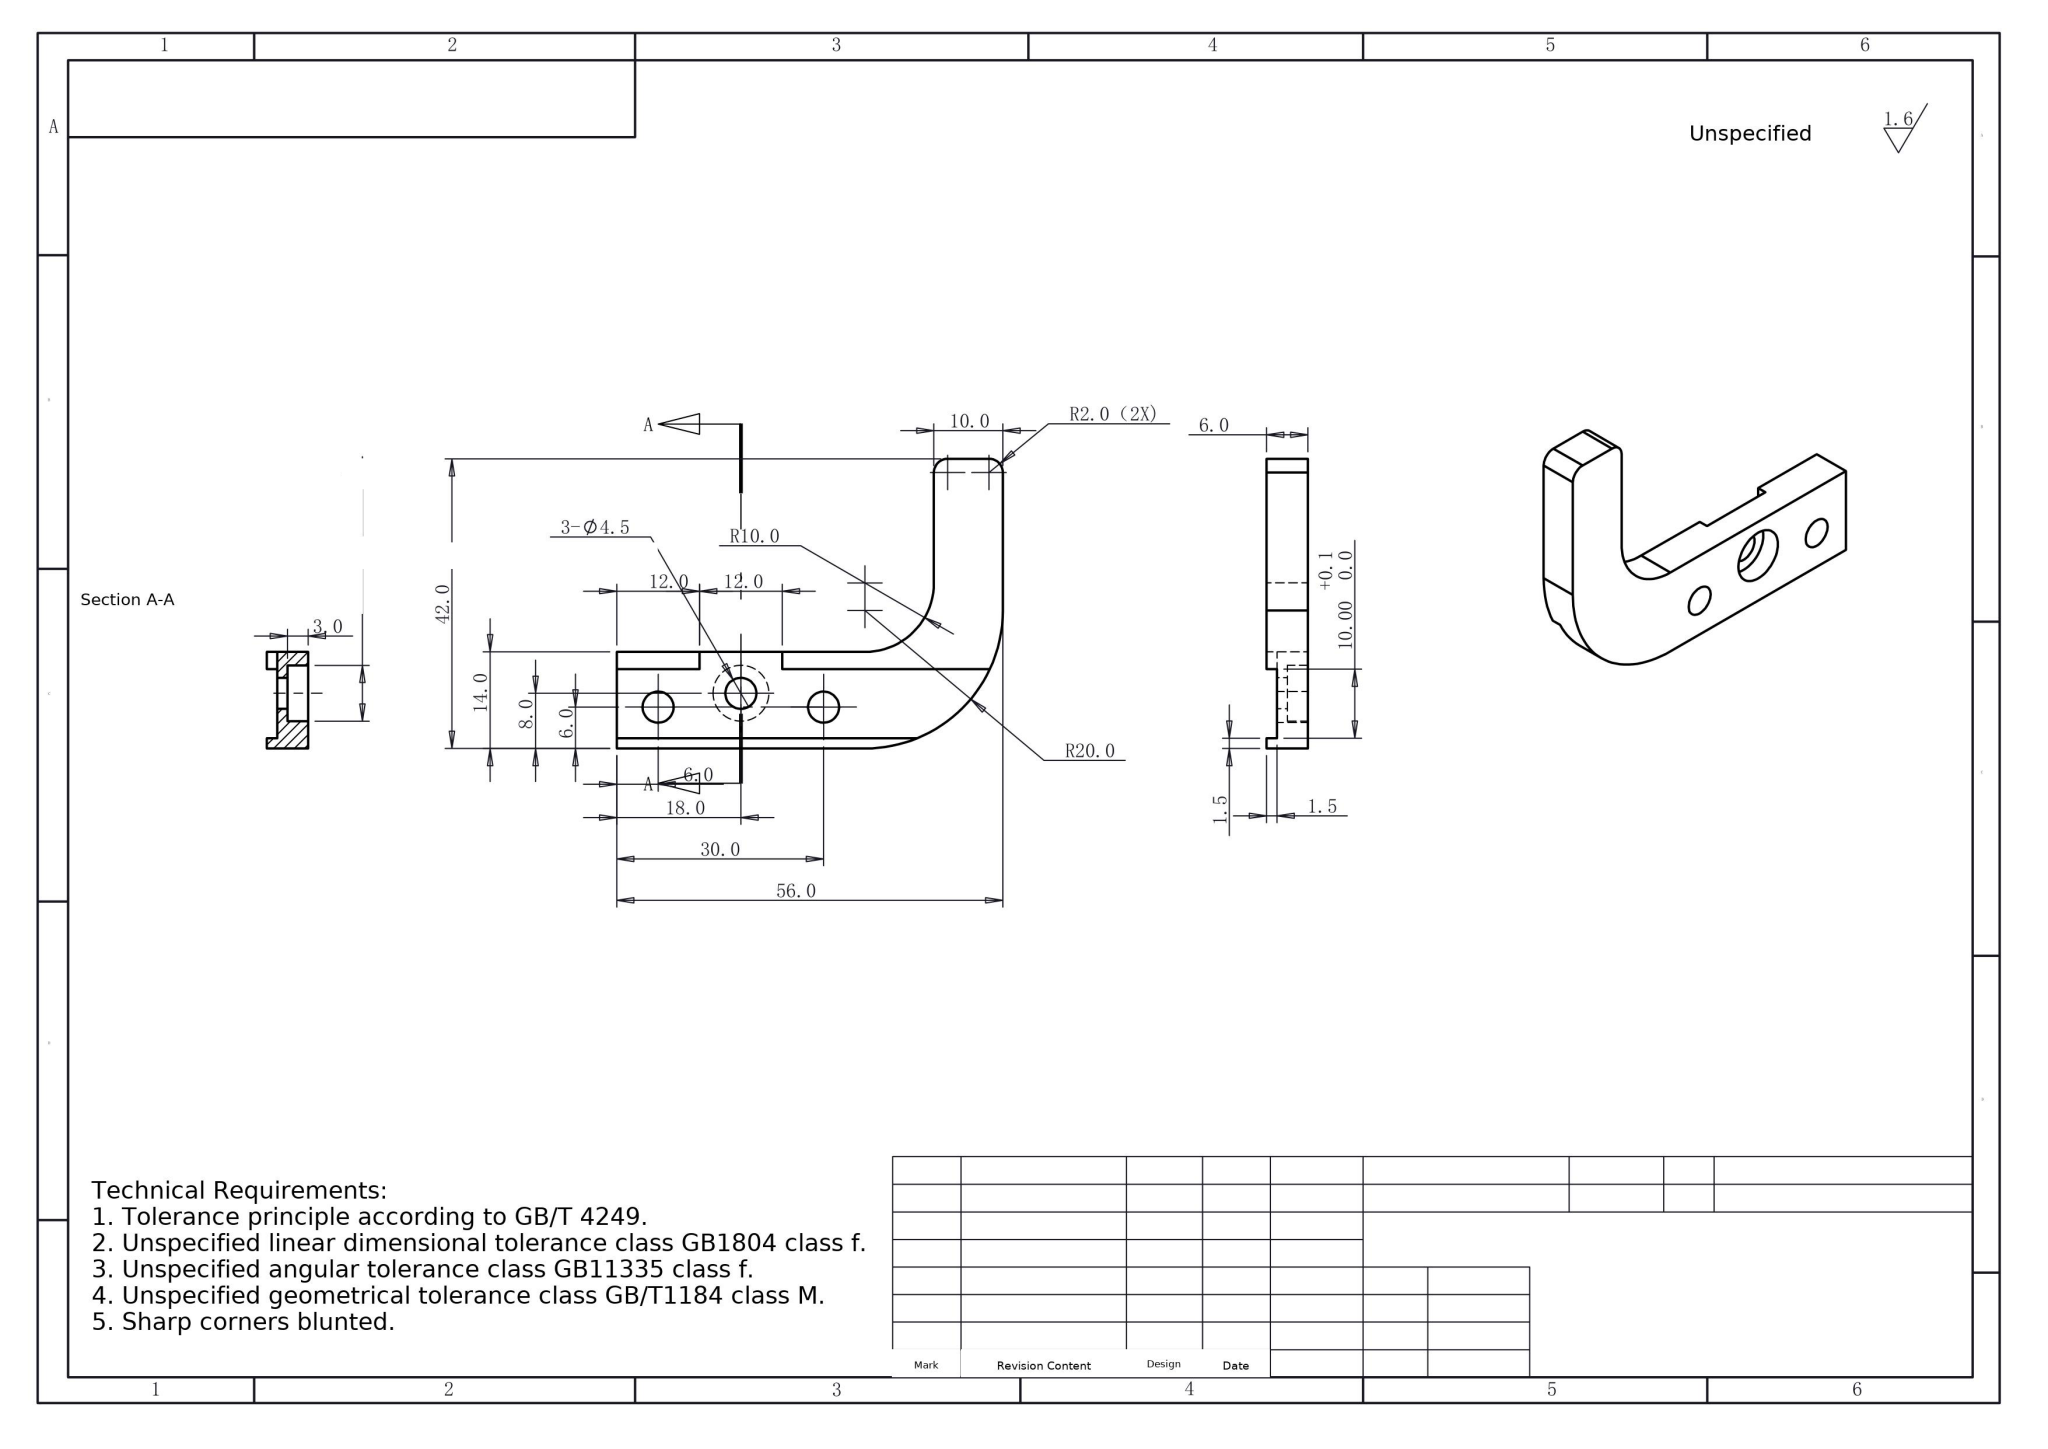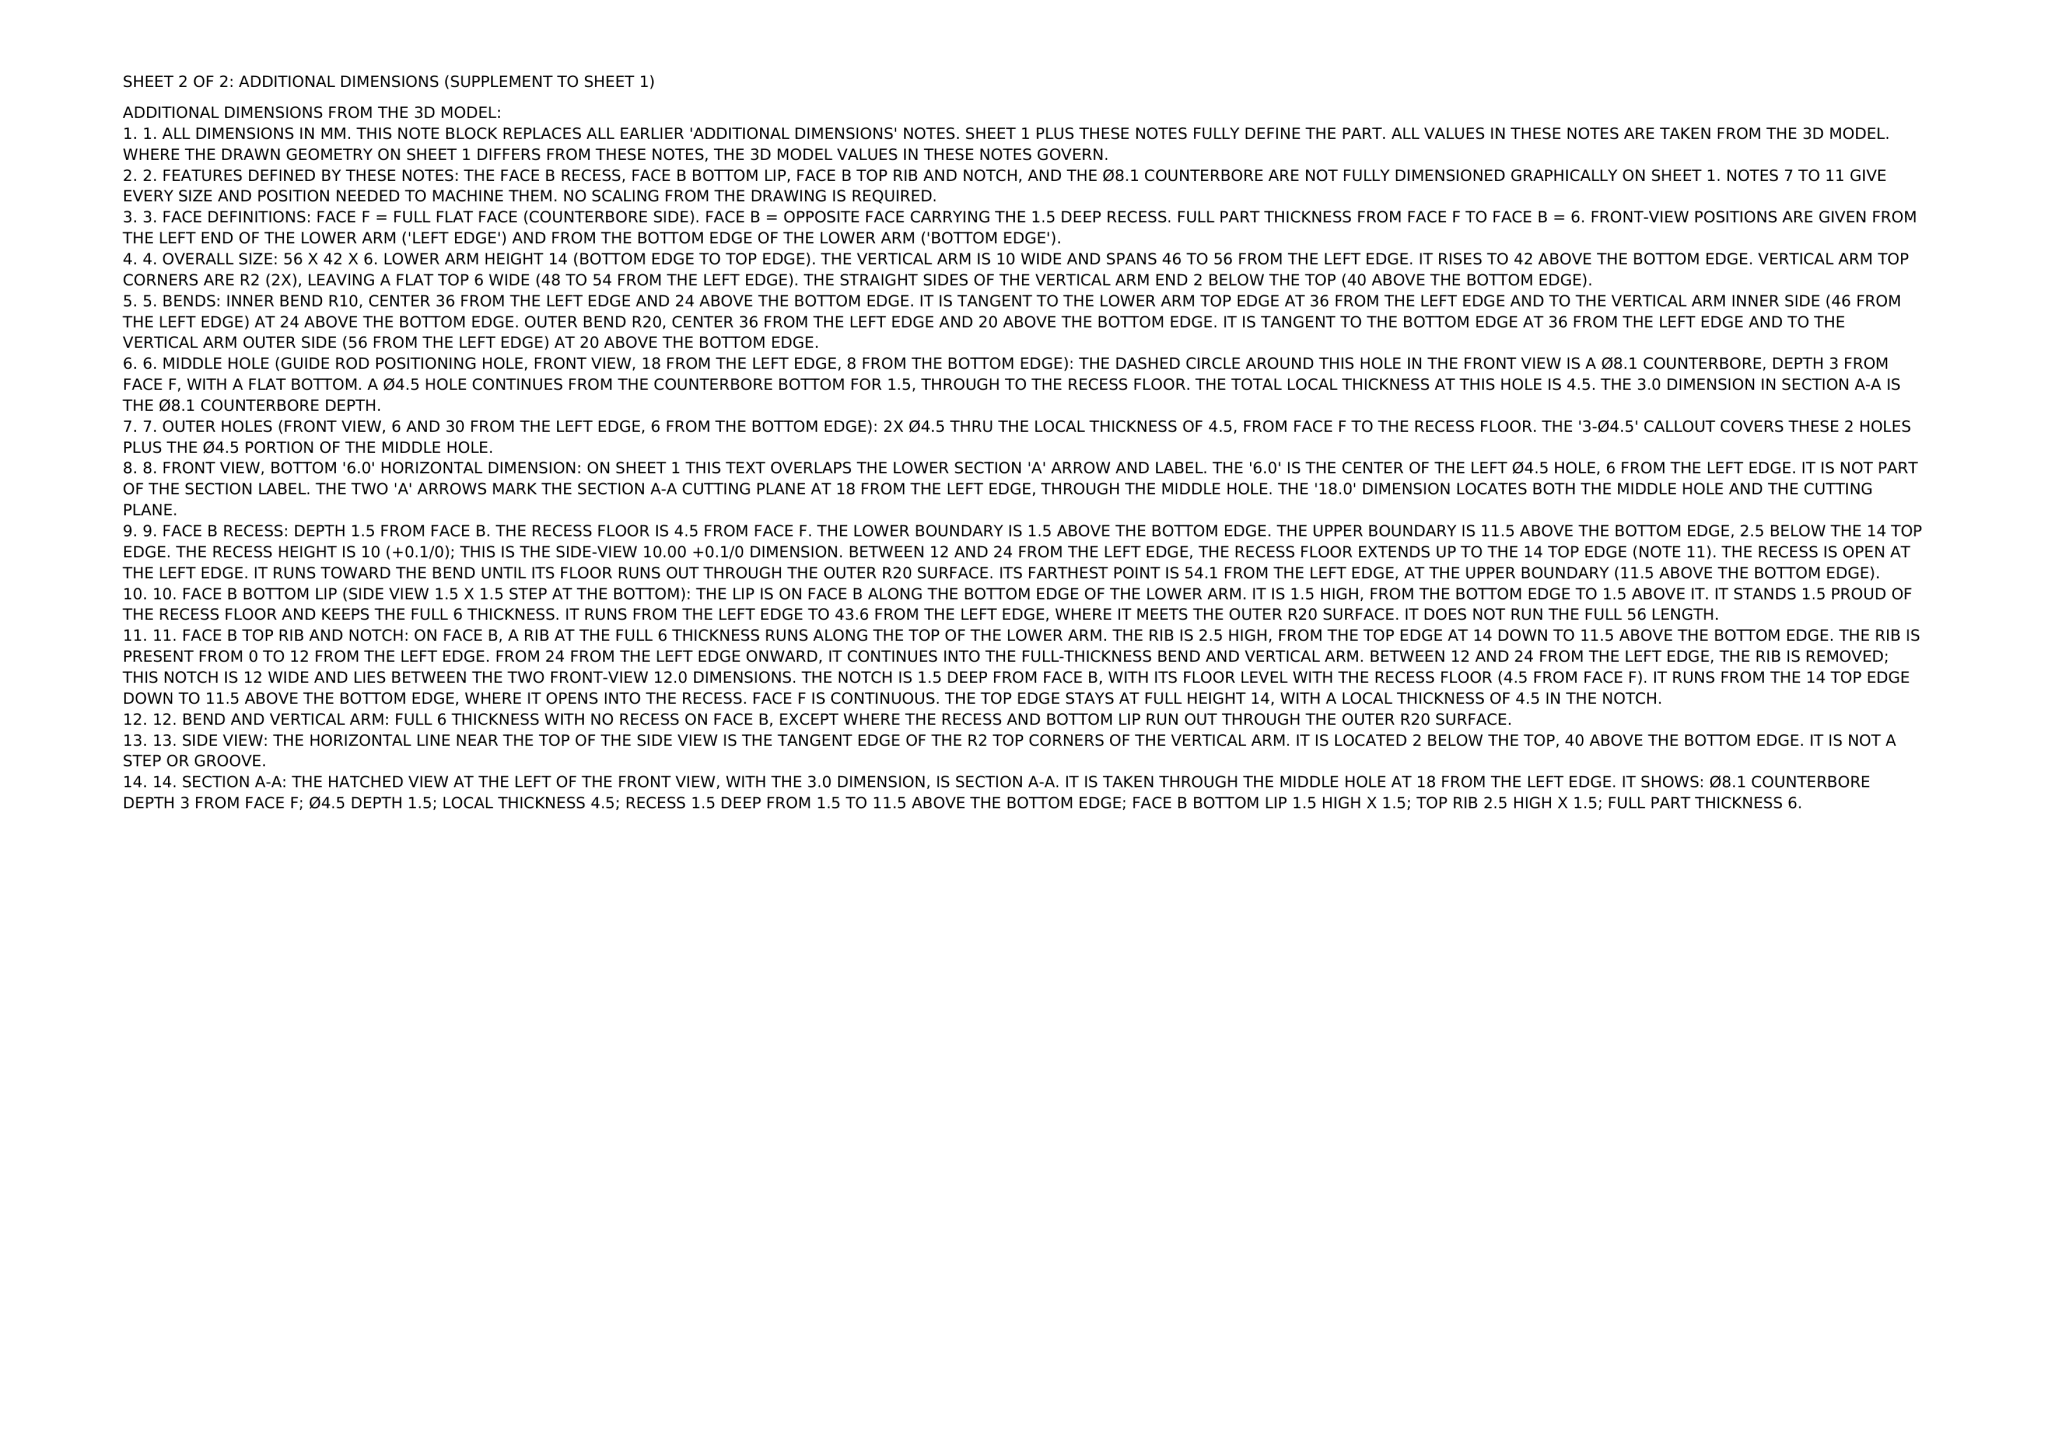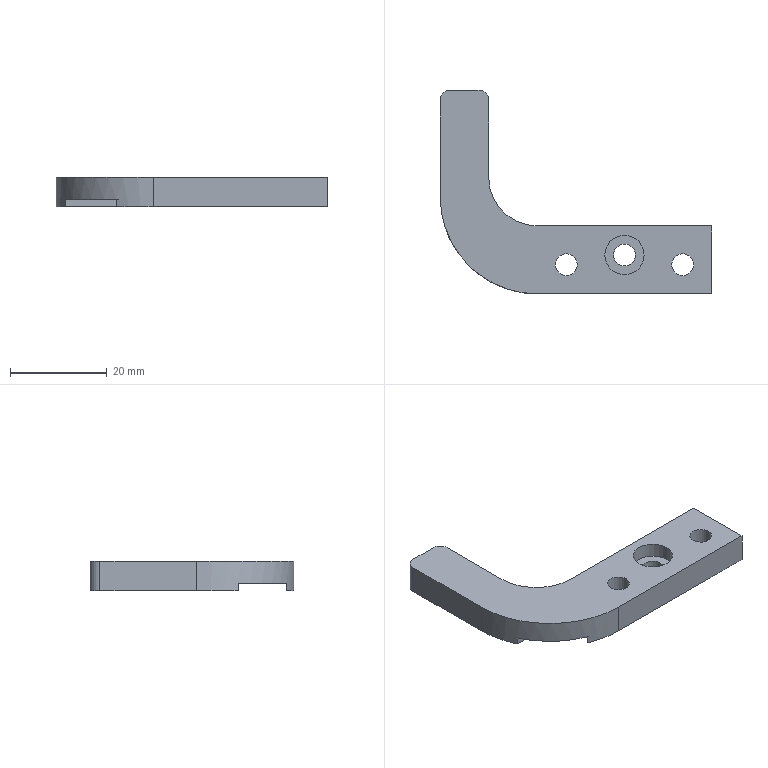Part | NX | mm | 1 solid | 29 faces | box 56 x 42 x 6 mm | volume 4868 mm3 | plane 17 | cylinder 12 | commonest cylinder face diameters 4.5 x6 8.1 x2 4 x2 20 x1 40 x1